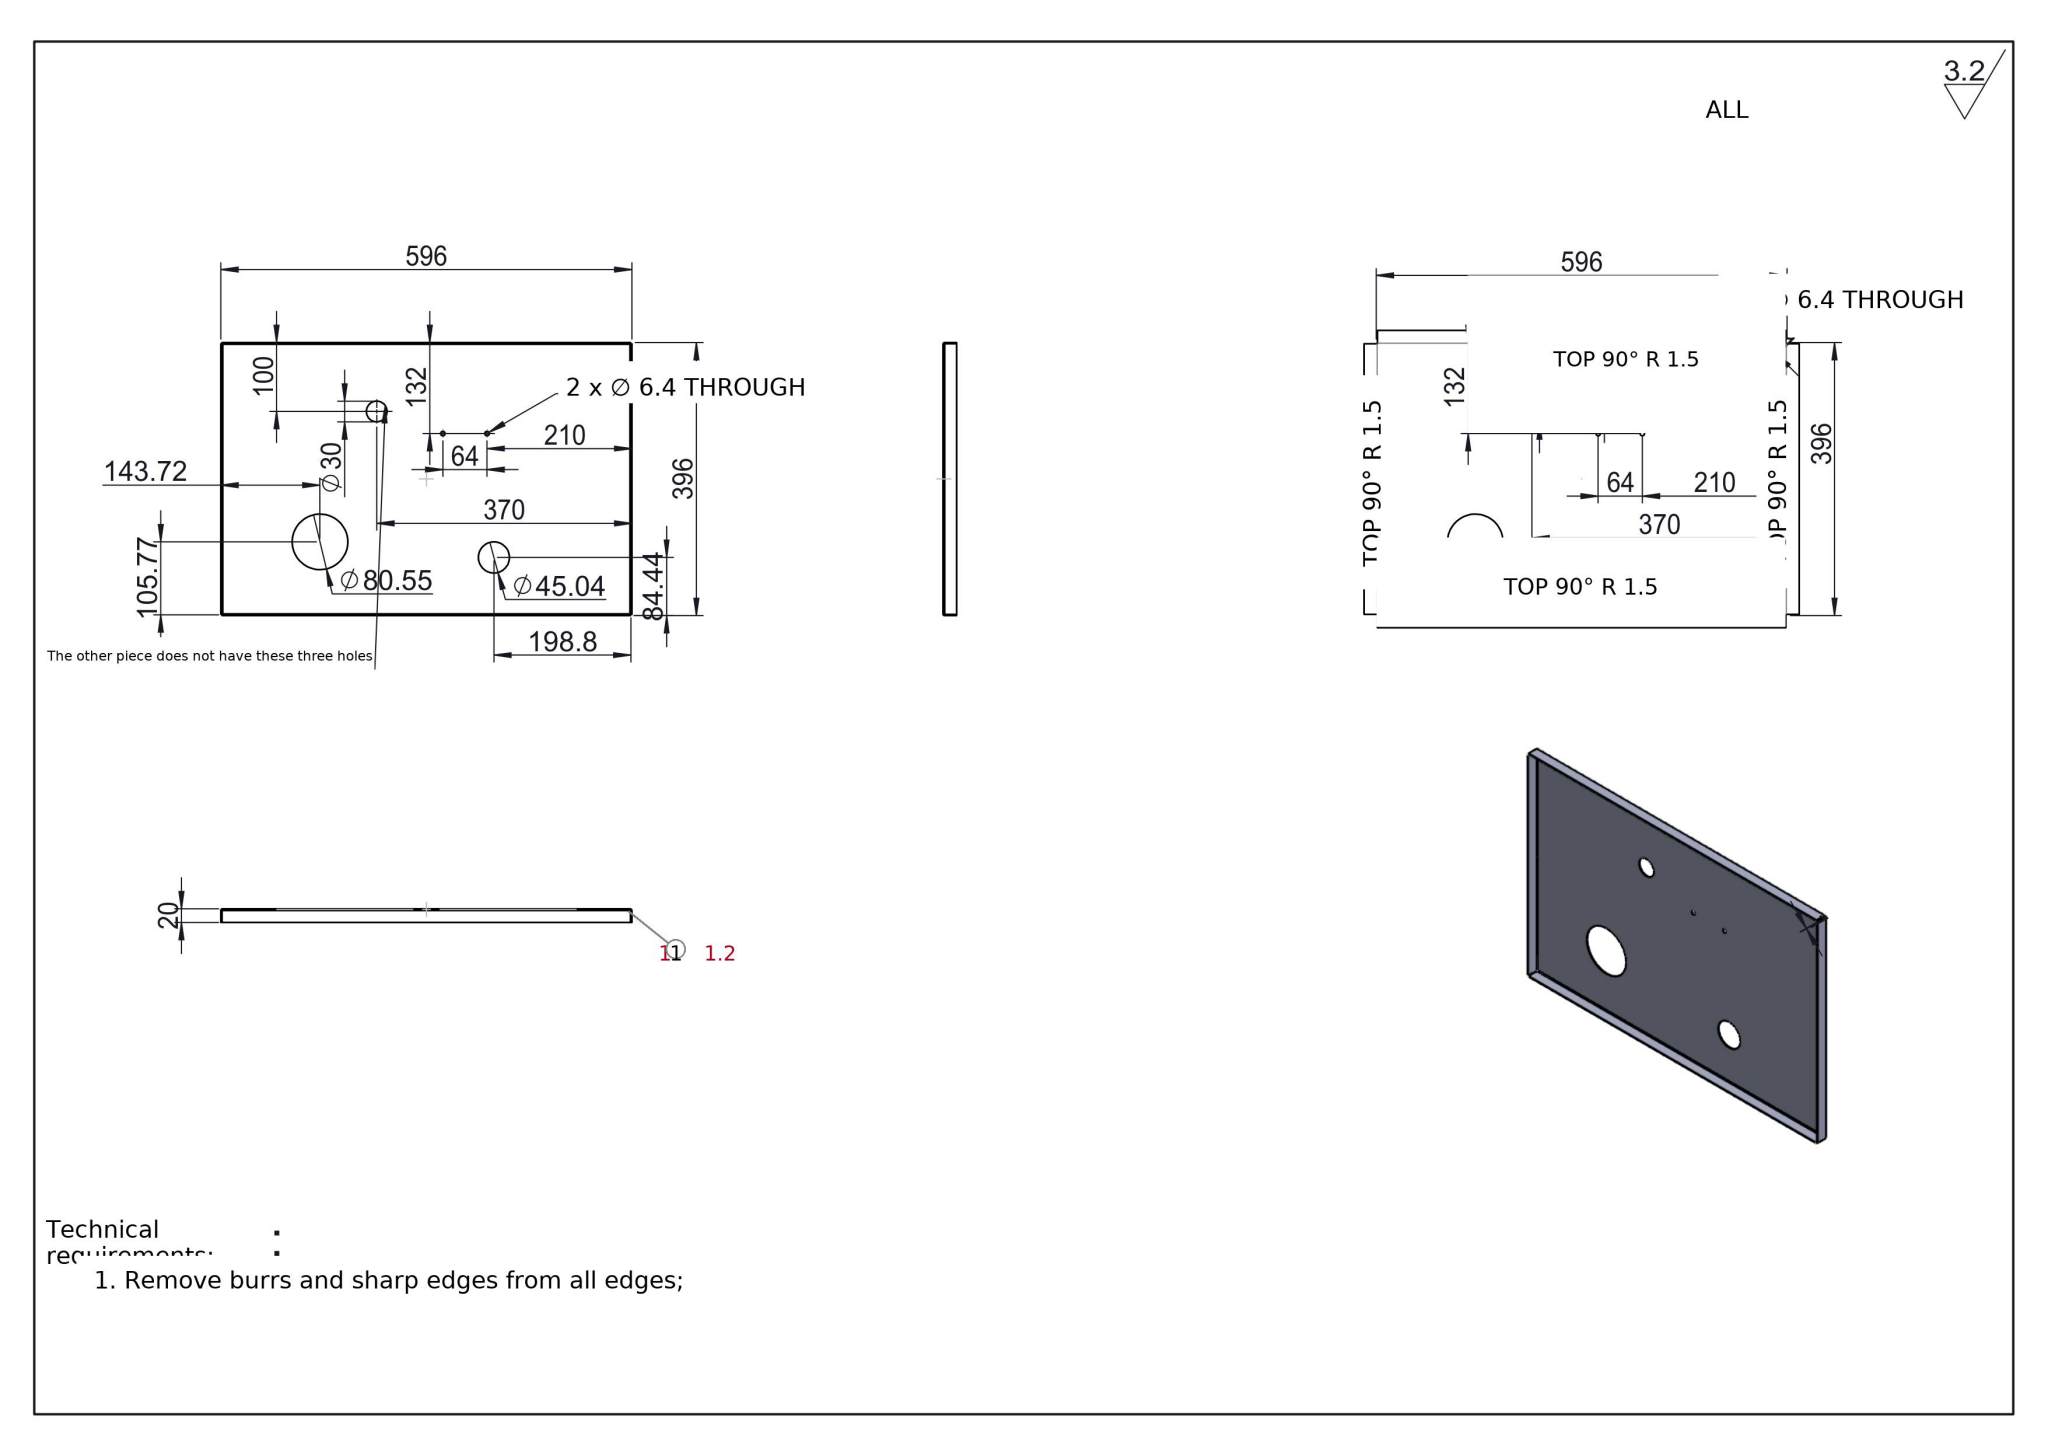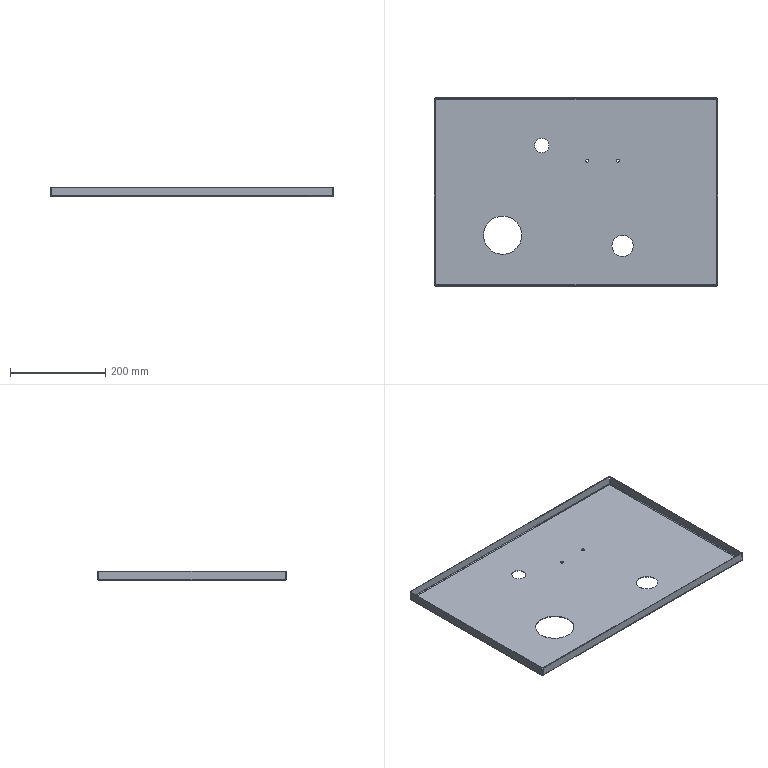Part | SolidWorks | mm | 1 solid | 48 faces | box 596 x 396 x 20 mm | volume 316525 mm3 | plane 22 | cylinder 18 | spline 8 | commonest cylinder face diameters 6.4 x4 5.4 x4 3 x4 45.045 x2 80.546 x2 30 x2